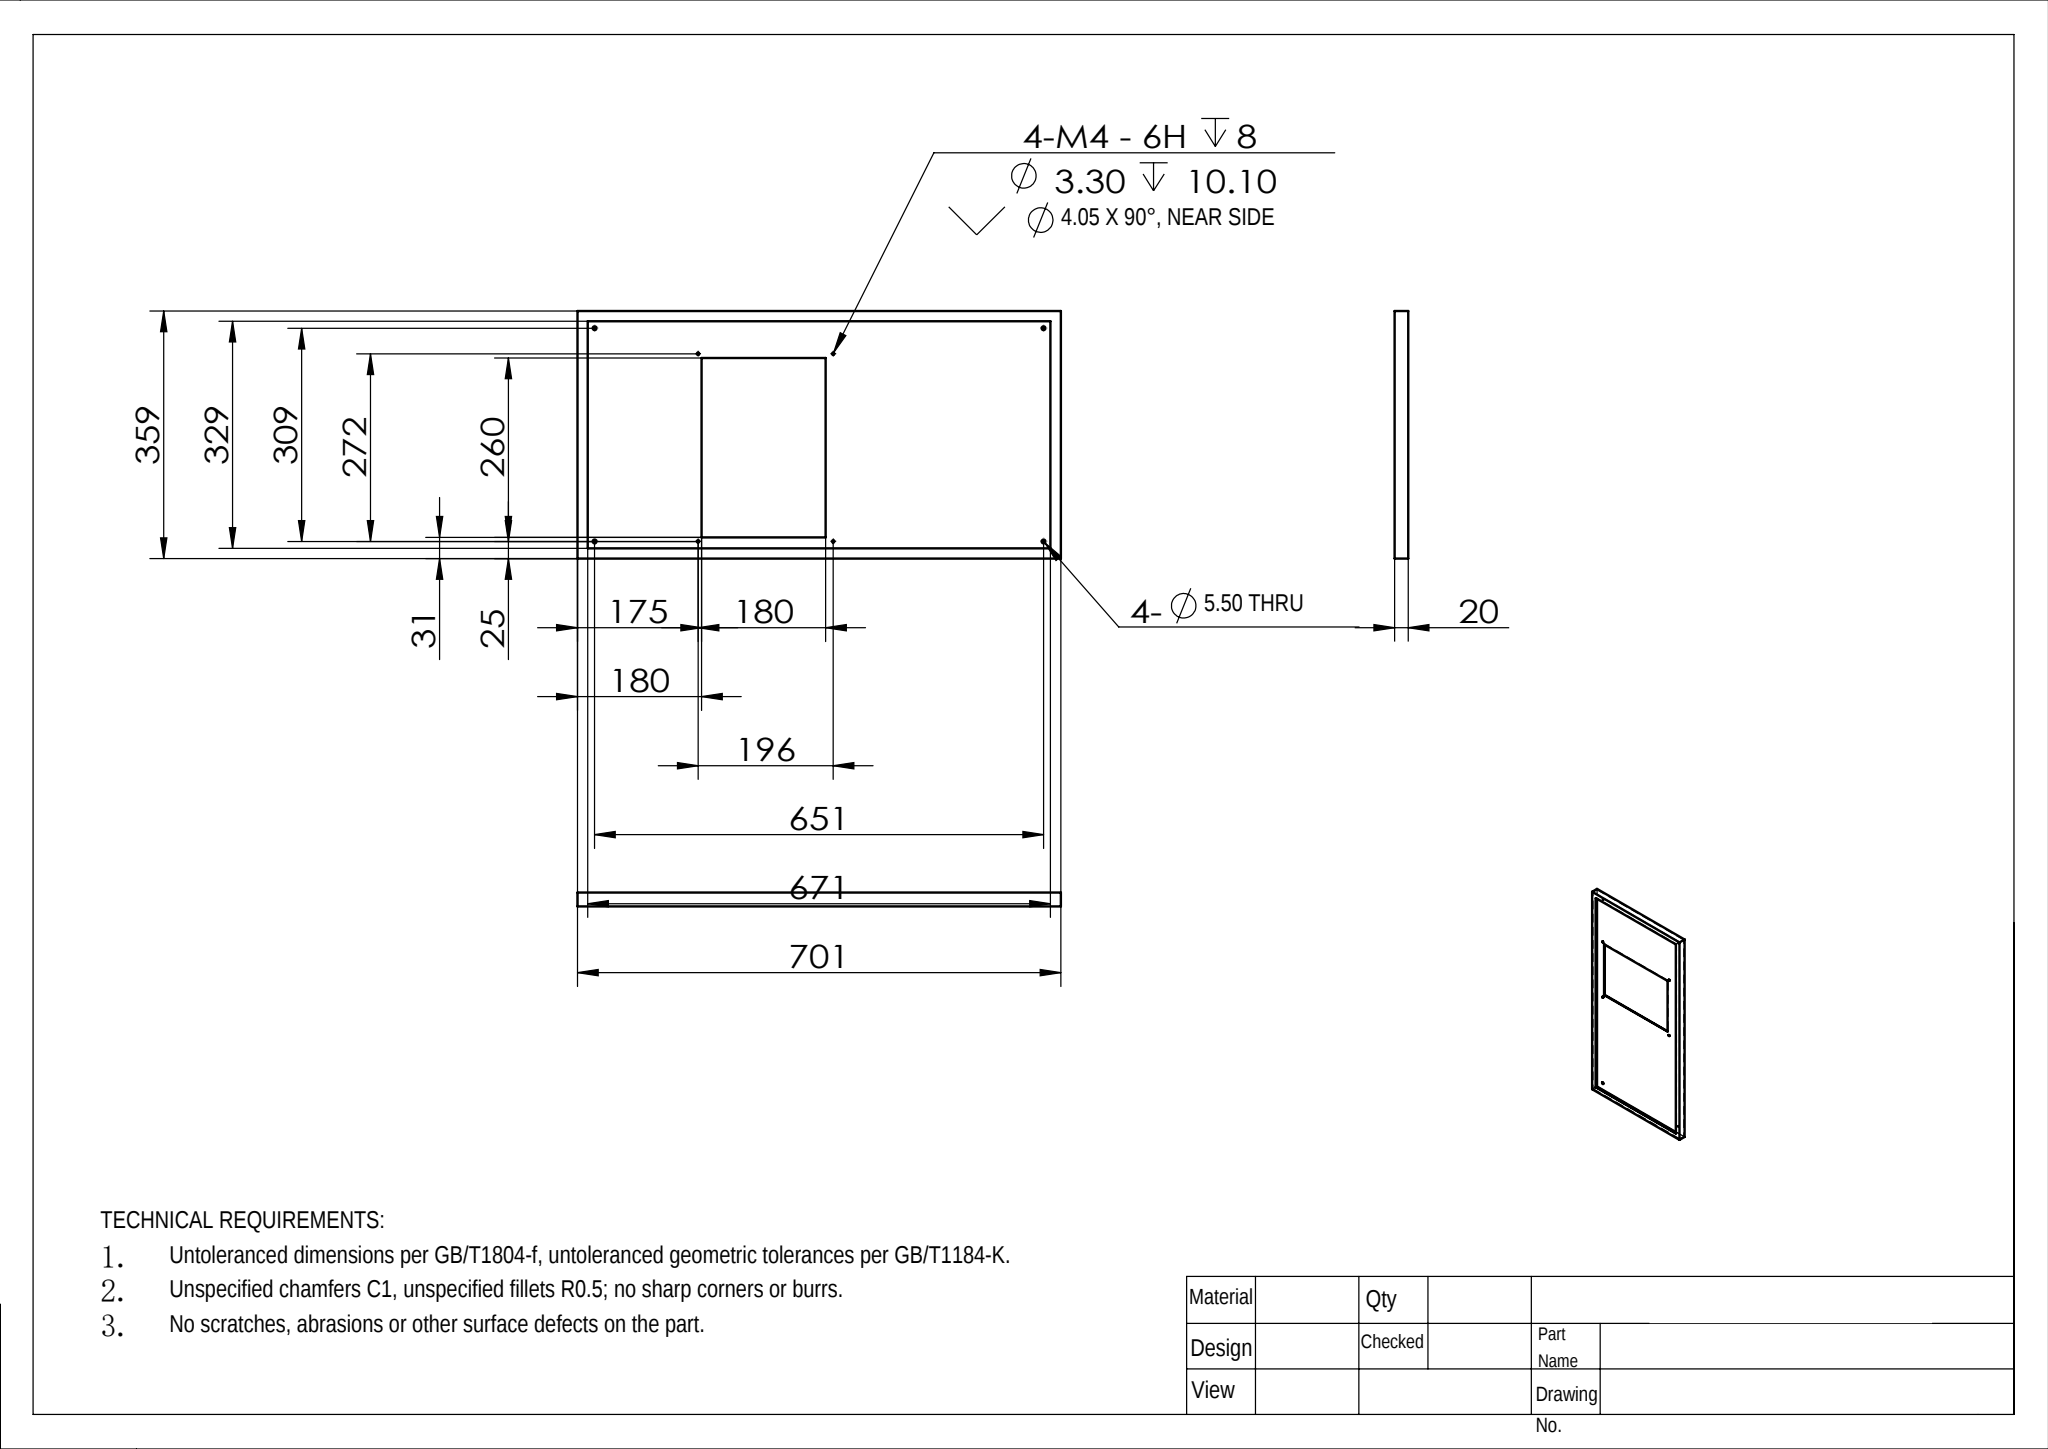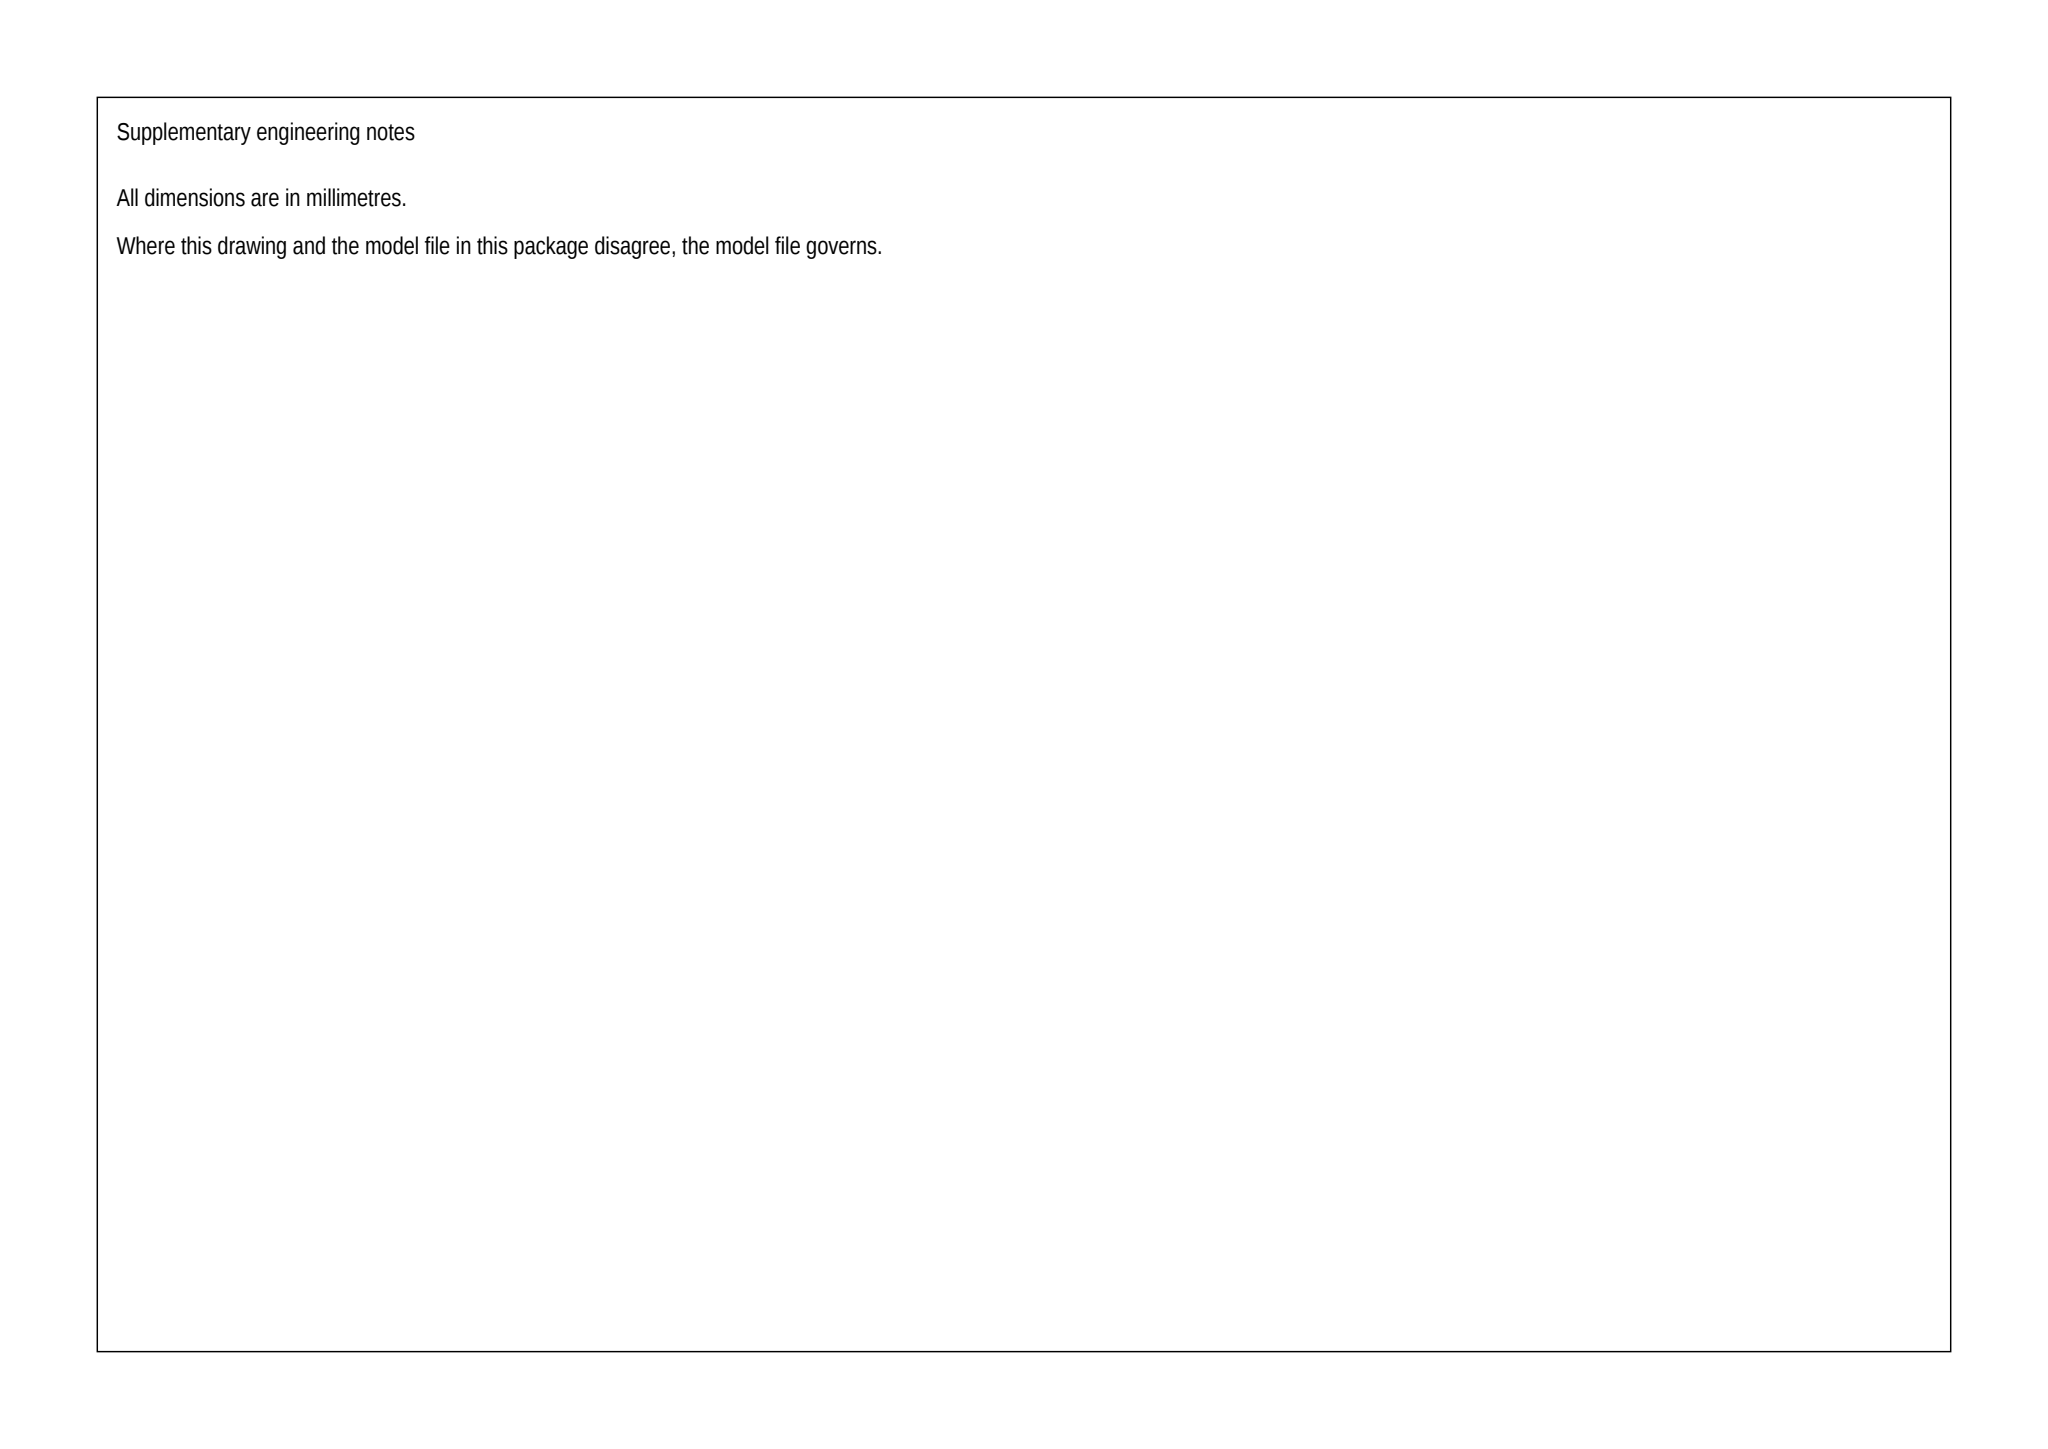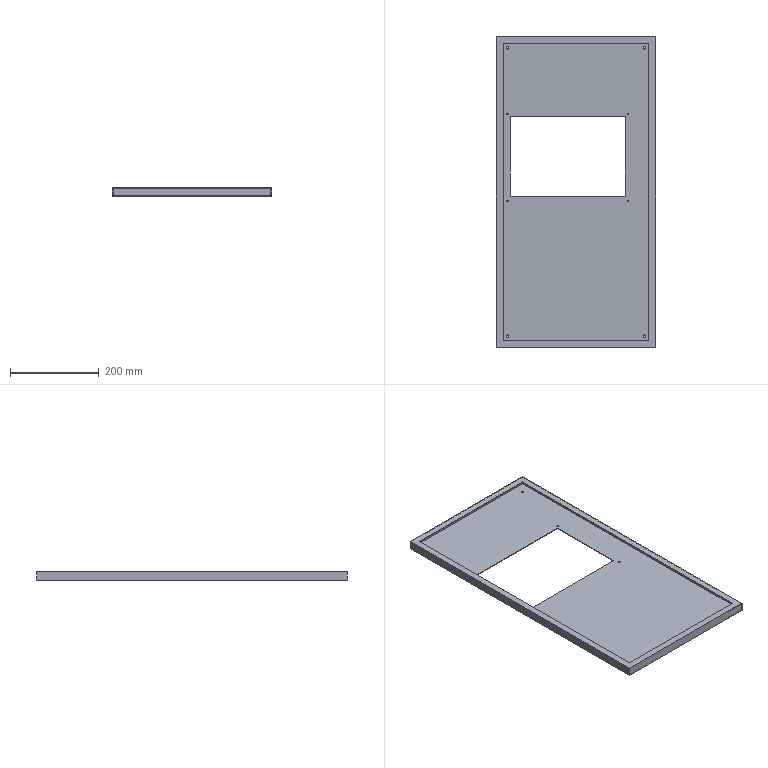Part | SolidWorks | mm | 1 solid | 44 faces | box 359 x 701 x 20 mm | volume 407348 mm3 | plane 20 | cylinder 16 | cone 8 | commonest cylinder face diameters 3.3 x8 5.5 x8
build123d program:
from build123d import *

# Parameters (mm, degrees)
SKETCH1_W                   = 359
SKETCH1_H                   = 701
BOSS_EXTRUDE1_DEPTH         = 20
SHELL2_T                    = -1.5
SKETCH11_R                  = 2.75
CUT_EXTRUDE6_DEPTH          = 788.834
SKETCH12_W                  = 359
SKETCH12_H                  = 701
SKETCH12_W_2                = 329
SKETCH12_H_2                = 671
BOSS_EXTRUDE2_DEPTH         = 1.5
M4_TAPPED_HOLE1_D           = 3.3
M4_TAPPED_HOLE1_DEPTH       = 10.1
M4_TAPPED_HOLE1_CSINK_D     = 4.05
M4_TAPPED_HOLE1_CSINK_ANGLE = 90
M4_TAPPED_HOLE1_TIP         = 0.9914
SKETCH15_W                  = 260
SKETCH15_H                  = 180
CUT_EXTRUDE7_DEPTH          = 10


with BuildPart() as part:
    # Sketch1 → Boss-Extrude1 (new body)
    with BuildSketch(Plane.XY):
        with Locations((179.5, 350.5)):
            Rectangle(SKETCH1_W, SKETCH1_H)
    extrude(amount=BOSS_EXTRUDE1_DEPTH)

    # Shell2
    shell2_openings = [part.faces().sort_by_distance(p)[0] for p in [
        (179.5, 350.5, 20),
    ]]
    offset(amount=SHELL2_T, openings=shell2_openings, kind=Kind.INTERSECTION)

    # Sketch11 → Cut-Extrude6 (cut, through all)
    with BuildSketch(Plane(origin=(0, 0, 0), x_dir=(-1, 0, 0), z_dir=(0, 0, -1))):
        with Locations((-25, 25)):
            Circle(SKETCH11_R)
        with Locations((-334, 25)):
            Circle(SKETCH11_R)
        with Locations((-334, 676)):
            Circle(SKETCH11_R)
        with Locations((-25, 676)):
            Circle(SKETCH11_R)
    extrude(amount=-CUT_EXTRUDE6_DEPTH, mode=Mode.SUBTRACT)

    # Sketch12 → Boss-Extrude2 (add)
    with BuildSketch(Plane.XY.offset(20)):
        with Locations((179.5, 350.5)):
            Rectangle(SKETCH12_W, SKETCH12_H)
        with Locations((179.5, 350.5)):
            Rectangle(SKETCH12_W_2, SKETCH12_H_2, mode=Mode.SUBTRACT)
    extrude(amount=-BOSS_EXTRUDE2_DEPTH)

    # M4 Tapped Hole1
    with Locations(Plane(origin=(0, 0, 0), x_dir=(-1, 0, 0), z_dir=(0, 0, -1))):
        with Locations((-25, 526), (-297, 526), (-25, 330), (-297, 330)):
            CounterSinkHole(M4_TAPPED_HOLE1_D / 2, M4_TAPPED_HOLE1_CSINK_D / 2, depth=M4_TAPPED_HOLE1_DEPTH, counter_sink_angle=M4_TAPPED_HOLE1_CSINK_ANGLE)
            with Locations((0, 0, -(M4_TAPPED_HOLE1_DEPTH + M4_TAPPED_HOLE1_TIP / 2))):  # 118° drill point
                Cone(0, M4_TAPPED_HOLE1_D / 2, M4_TAPPED_HOLE1_TIP, mode=Mode.SUBTRACT)

    # Sketch15 → Cut-Extrude7 (cut)
    with BuildSketch(Plane(origin=(0, 0, 0), x_dir=(-1, 0, 0), z_dir=(0, 0, -1))):
        with Locations((-161, 431)):
            Rectangle(SKETCH15_W, SKETCH15_H)
    extrude(amount=-CUT_EXTRUDE7_DEPTH, mode=Mode.SUBTRACT)


solid = part.part